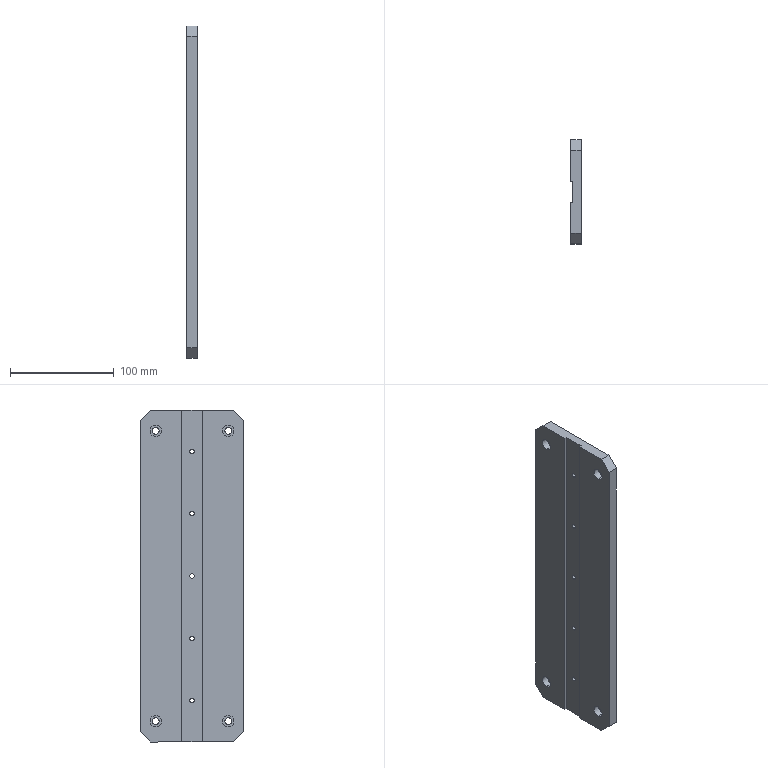Component | SolidWorks | SidePlate-2 | 1 solid | 44 faces | box 10.02 x 100 x 320 mm | volume 301720 mm3 | cylinder 26 | plane 18 | commonest cylinder face diameters 4.2 x10 11 x8 6.6 x8
build123d program:
from build123d import *

# Parameters (mm, degrees)
SKETCH1_W                                       = 320
SKETCH1_H                                       = 100
BOSS_EXTRUDE1_DEPTH                             = 10
CHAMFER1_SIZE                                   = 10
M6_HEX_SOCKET_HEAD_CAP_SCREW_CBORE1_D           = 6.6
M6_HEX_SOCKET_HEAD_CAP_SCREW_CBORE1_CBORE_D     = 11
M6_HEX_SOCKET_HEAD_CAP_SCREW_CBORE1_CBORE_DEPTH = 6.4
M5_TAPPED_HOLE1_D                               = 4.2
SKETCH7_W                                       = 320
SKETCH7_H                                       = 20
CUT_EXTRUDE1_DEPTH                              = 2


with BuildPart() as part:
    # Sketch1 → Boss-Extrude1 (new body)
    with BuildSketch(Plane.XY):
        Rectangle(SKETCH1_W, SKETCH1_H)
    extrude(amount=BOSS_EXTRUDE1_DEPTH)

    # Chamfer1
    chamfer1_edges = [part.edges().sort_by_distance(p)[0] for p in [
        (-160, 50, 5),
        (160, 50, 5),
        (160, -50, 5),
        (-160, -50, 5),
    ]]
    chamfer(chamfer1_edges, length=CHAMFER1_SIZE)

    # M6 Hex Socket Head Cap Screw CBORE1 (through all)
    with Locations(Plane.XY.offset(10)):
        with Locations((-140, 35), (-140, -35), (140, 35), (140, -35)):
            CounterBoreHole(M6_HEX_SOCKET_HEAD_CAP_SCREW_CBORE1_D / 2, M6_HEX_SOCKET_HEAD_CAP_SCREW_CBORE1_CBORE_D / 2, M6_HEX_SOCKET_HEAD_CAP_SCREW_CBORE1_CBORE_DEPTH)

    # M5 Tapped Hole1 (through all)
    with Locations(Plane.XY.offset(10)):
        with Locations((0, 0), (-60, 0), (-120, 0), (60, 0), (120, 0)):
            Hole(M5_TAPPED_HOLE1_D / 2)

    # Sketch7 → Cut-Extrude1 (cut)
    with BuildSketch(Plane.XY.offset(10)):
        Rectangle(SKETCH7_W, SKETCH7_H)
    extrude(amount=-CUT_EXTRUDE1_DEPTH, mode=Mode.SUBTRACT)


solid = part.part

# Placed as in the assembly
solid = solid.moved(Location((1994.163, 3833.765, 1079.241), (0, -90, 0)))